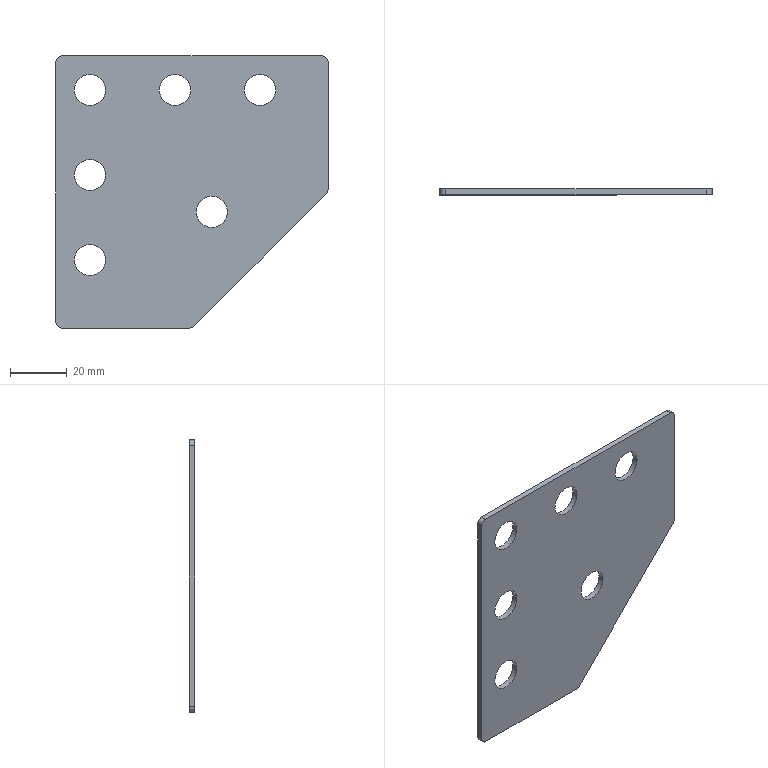Component | SolidWorks | Assembly2-1_Stiffener-2 | 1 solid | 24 faces | box 96 x 2 x 96 mm | volume 14982 mm3 | cylinder 17 | plane 7 | commonest cylinder face diameters 11 x12 4 x5
STEP:
#1=COLOUR_RGB('',0.7922,0.8196,0.9333);
#2=FILL_AREA_STYLE_COLOUR('',#1);
#3=FILL_AREA_STYLE('',(#2));
#4=SURFACE_STYLE_FILL_AREA(#3);
#5=SURFACE_SIDE_STYLE('',(#4));
#6=SURFACE_STYLE_USAGE(.BOTH.,#5);
#7=PRESENTATION_STYLE_ASSIGNMENT((#6));
#8=CARTESIAN_POINT('',(-2.167,43.439,0.3839));
#9=VERTEX_POINT('',#8);
#10=CARTESIAN_POINT('',(-1.733,43.439,0.3839));
#11=VERTEX_POINT('',#10);
#12=CARTESIAN_POINT('',(-1.95,43.439,0.3839));
#13=DIRECTION('',(-0.,1.,0.));
#14=DIRECTION('',(1.,0.,-0.));
#15=AXIS2_PLACEMENT_3D('',#12,#13,#14);
#16=CIRCLE('',#15,0.2165);
#17=EDGE_CURVE('',#9,#11,#16,.T.);
#18=ORIENTED_EDGE('',*,*,#17,.F.);
#19=CARTESIAN_POINT('',(-2.167,43.517,0.3839));
#20=VERTEX_POINT('',#19);
#21=CARTESIAN_POINT('',(-2.167,43.124,0.3839));
#22=DIRECTION('',(-0.,1.,0.));
#23=VECTOR('',#22,39.37);
#24=LINE('',#21,#23);
#25=EDGE_CURVE('',#9,#20,#24,.T.);
#26=ORIENTED_EDGE('',*,*,#25,.T.);
#27=CARTESIAN_POINT('',(-1.733,43.517,0.3839));
#28=VERTEX_POINT('',#27);
#29=CARTESIAN_POINT('',(-1.95,43.517,0.3839));
#30=DIRECTION('',(-0.,1.,0.));
#31=DIRECTION('',(1.,0.,-0.));
#32=AXIS2_PLACEMENT_3D('',#29,#30,#31);
#33=CIRCLE('',#32,0.2165);
#34=EDGE_CURVE('',#20,#28,#33,.T.);
#35=ORIENTED_EDGE('',*,*,#34,.T.);
#36=CARTESIAN_POINT('',(-1.733,43.124,0.3839));
#37=DIRECTION('',(-0.,1.,0.));
#38=VECTOR('',#37,39.37);
#39=LINE('',#36,#38);
#40=EDGE_CURVE('',#11,#28,#39,.T.);
#41=ORIENTED_EDGE('',*,*,#40,.F.);
#42=EDGE_LOOP('',(#18,#26,#35,#41));
#43=FACE_OUTER_BOUND('',#42,.T.);
#44=CARTESIAN_POINT('',(-1.95,43.124,0.3839));
#45=DIRECTION('',(-0.,1.,0.));
#46=DIRECTION('',(1.,0.,-0.));
#47=AXIS2_PLACEMENT_3D('',#44,#45,#46);
#48=CYLINDRICAL_SURFACE('',#47,0.2165);
#49=ADVANCED_FACE('',(#43),#48,.F.);
#50=CARTESIAN_POINT('',(-3.859,43.439,-0.2854));
#51=VERTEX_POINT('',#50);
#52=CARTESIAN_POINT('',(-3.426,43.439,-0.2854));
#53=VERTEX_POINT('',#52);
#54=CARTESIAN_POINT('',(-3.643,43.439,-0.2854));
#55=DIRECTION('',(-0.,1.,0.));
#56=DIRECTION('',(1.,0.,-0.));
#57=AXIS2_PLACEMENT_3D('',#54,#55,#56);
#58=CIRCLE('',#57,0.2165);
#59=EDGE_CURVE('',#51,#53,#58,.T.);
#60=ORIENTED_EDGE('',*,*,#59,.F.);
#61=CARTESIAN_POINT('',(-3.859,43.517,-0.2854));
#62=VERTEX_POINT('',#61);
#63=CARTESIAN_POINT('',(-3.859,43.124,-0.2854));
#64=DIRECTION('',(-0.,1.,0.));
#65=VECTOR('',#64,39.37);
#66=LINE('',#63,#65);
#67=EDGE_CURVE('',#51,#62,#66,.T.);
#68=ORIENTED_EDGE('',*,*,#67,.T.);
#69=CARTESIAN_POINT('',(-3.426,43.517,-0.2854));
#70=VERTEX_POINT('',#69);
#71=CARTESIAN_POINT('',(-3.643,43.517,-0.2854));
#72=DIRECTION('',(-0.,1.,0.));
#73=DIRECTION('',(1.,0.,-0.));
#74=AXIS2_PLACEMENT_3D('',#71,#72,#73);
#75=CIRCLE('',#74,0.2165);
#76=EDGE_CURVE('',#62,#70,#75,.T.);
#77=ORIENTED_EDGE('',*,*,#76,.T.);
#78=CARTESIAN_POINT('',(-3.426,43.124,-0.2854));
#79=DIRECTION('',(-0.,1.,0.));
#80=VECTOR('',#79,39.37);
#81=LINE('',#78,#80);
#82=EDGE_CURVE('',#53,#70,#81,.T.);
#83=ORIENTED_EDGE('',*,*,#82,.F.);
#84=EDGE_LOOP('',(#60,#68,#77,#83));
#85=FACE_OUTER_BOUND('',#84,.T.);
#86=CARTESIAN_POINT('',(-3.643,43.124,-0.2854));
#87=DIRECTION('',(-0.,1.,0.));
#88=DIRECTION('',(1.,0.,-0.));
#89=AXIS2_PLACEMENT_3D('',#86,#87,#88);
#90=CYLINDRICAL_SURFACE('',#89,0.2165);
#91=ADVANCED_FACE('',(#85),#90,.F.);
#92=CARTESIAN_POINT('',(-3.859,43.439,0.8957));
#93=VERTEX_POINT('',#92);
#94=CARTESIAN_POINT('',(-3.426,43.439,0.8957));
#95=VERTEX_POINT('',#94);
#96=CARTESIAN_POINT('',(-3.643,43.439,0.8957));
#97=DIRECTION('',(-0.,1.,0.));
#98=DIRECTION('',(1.,0.,-0.));
#99=AXIS2_PLACEMENT_3D('',#96,#97,#98);
#100=CIRCLE('',#99,0.2165);
#101=EDGE_CURVE('',#93,#95,#100,.T.);
#102=ORIENTED_EDGE('',*,*,#101,.F.);
#103=CARTESIAN_POINT('',(-3.859,43.517,0.8957));
#104=VERTEX_POINT('',#103);
#105=CARTESIAN_POINT('',(-3.859,43.124,0.8957));
#106=DIRECTION('',(-0.,1.,0.));
#107=VECTOR('',#106,39.37);
#108=LINE('',#105,#107);
#109=EDGE_CURVE('',#93,#104,#108,.T.);
#110=ORIENTED_EDGE('',*,*,#109,.T.);
#111=CARTESIAN_POINT('',(-3.426,43.517,0.8957));
#112=VERTEX_POINT('',#111);
#113=CARTESIAN_POINT('',(-3.643,43.517,0.8957));
#114=DIRECTION('',(-0.,1.,0.));
#115=DIRECTION('',(1.,0.,-0.));
#116=AXIS2_PLACEMENT_3D('',#113,#114,#115);
#117=CIRCLE('',#116,0.2165);
#118=EDGE_CURVE('',#104,#112,#117,.T.);
#119=ORIENTED_EDGE('',*,*,#118,.T.);
#120=CARTESIAN_POINT('',(-3.426,43.124,0.8957));
#121=DIRECTION('',(-0.,1.,0.));
#122=VECTOR('',#121,39.37);
#123=LINE('',#120,#122);
#124=EDGE_CURVE('',#95,#112,#123,.T.);
#125=ORIENTED_EDGE('',*,*,#124,.F.);
#126=EDGE_LOOP('',(#102,#110,#119,#125));
#127=FACE_OUTER_BOUND('',#126,.T.);
#128=CARTESIAN_POINT('',(-3.643,43.124,0.8957));
#129=DIRECTION('',(-0.,1.,0.));
#130=DIRECTION('',(1.,0.,-0.));
#131=AXIS2_PLACEMENT_3D('',#128,#129,#130);
#132=CYLINDRICAL_SURFACE('',#131,0.2165);
#133=ADVANCED_FACE('',(#127),#132,.F.);
#134=CARTESIAN_POINT('',(-1.497,43.439,2.077));
#135=VERTEX_POINT('',#134);
#136=CARTESIAN_POINT('',(-1.064,43.439,2.077));
#137=VERTEX_POINT('',#136);
#138=CARTESIAN_POINT('',(-1.281,43.439,2.077));
#139=DIRECTION('',(-0.,1.,0.));
#140=DIRECTION('',(1.,0.,-0.));
#141=AXIS2_PLACEMENT_3D('',#138,#139,#140);
#142=CIRCLE('',#141,0.2165);
#143=EDGE_CURVE('',#135,#137,#142,.T.);
#144=ORIENTED_EDGE('',*,*,#143,.F.);
#145=CARTESIAN_POINT('',(-1.497,43.517,2.077));
#146=VERTEX_POINT('',#145);
#147=CARTESIAN_POINT('',(-1.497,43.124,2.077));
#148=DIRECTION('',(-0.,1.,0.));
#149=VECTOR('',#148,39.37);
#150=LINE('',#147,#149);
#151=EDGE_CURVE('',#135,#146,#150,.T.);
#152=ORIENTED_EDGE('',*,*,#151,.T.);
#153=CARTESIAN_POINT('',(-1.064,43.517,2.077));
#154=VERTEX_POINT('',#153);
#155=CARTESIAN_POINT('',(-1.281,43.517,2.077));
#156=DIRECTION('',(-0.,1.,0.));
#157=DIRECTION('',(1.,0.,-0.));
#158=AXIS2_PLACEMENT_3D('',#155,#156,#157);
#159=CIRCLE('',#158,0.2165);
#160=EDGE_CURVE('',#146,#154,#159,.T.);
#161=ORIENTED_EDGE('',*,*,#160,.T.);
#162=CARTESIAN_POINT('',(-1.064,43.124,2.077));
#163=DIRECTION('',(-0.,1.,0.));
#164=VECTOR('',#163,39.37);
#165=LINE('',#162,#164);
#166=EDGE_CURVE('',#137,#154,#165,.T.);
#167=ORIENTED_EDGE('',*,*,#166,.F.);
#168=EDGE_LOOP('',(#144,#152,#161,#167));
#169=FACE_OUTER_BOUND('',#168,.T.);
#170=CARTESIAN_POINT('',(-1.281,43.124,2.077));
#171=DIRECTION('',(-0.,1.,0.));
#172=DIRECTION('',(1.,0.,-0.));
#173=AXIS2_PLACEMENT_3D('',#170,#171,#172);
#174=CYLINDRICAL_SURFACE('',#173,0.2165);
#175=ADVANCED_FACE('',(#169),#174,.F.);
#176=CARTESIAN_POINT('',(-2.678,43.439,2.077));
#177=VERTEX_POINT('',#176);
#178=CARTESIAN_POINT('',(-2.245,43.439,2.077));
#179=VERTEX_POINT('',#178);
#180=CARTESIAN_POINT('',(-2.462,43.439,2.077));
#181=DIRECTION('',(-0.,1.,0.));
#182=DIRECTION('',(1.,0.,-0.));
#183=AXIS2_PLACEMENT_3D('',#180,#181,#182);
#184=CIRCLE('',#183,0.2165);
#185=EDGE_CURVE('',#177,#179,#184,.T.);
#186=ORIENTED_EDGE('',*,*,#185,.F.);
#187=CARTESIAN_POINT('',(-2.678,43.517,2.077));
#188=VERTEX_POINT('',#187);
#189=CARTESIAN_POINT('',(-2.678,43.124,2.077));
#190=DIRECTION('',(-0.,1.,0.));
#191=VECTOR('',#190,39.37);
#192=LINE('',#189,#191);
#193=EDGE_CURVE('',#177,#188,#192,.T.);
#194=ORIENTED_EDGE('',*,*,#193,.T.);
#195=CARTESIAN_POINT('',(-2.245,43.517,2.077));
#196=VERTEX_POINT('',#195);
#197=CARTESIAN_POINT('',(-2.462,43.517,2.077));
#198=DIRECTION('',(-0.,1.,0.));
#199=DIRECTION('',(1.,0.,-0.));
#200=AXIS2_PLACEMENT_3D('',#197,#198,#199);
#201=CIRCLE('',#200,0.2165);
#202=EDGE_CURVE('',#188,#196,#201,.T.);
#203=ORIENTED_EDGE('',*,*,#202,.T.);
#204=CARTESIAN_POINT('',(-2.245,43.124,2.077));
#205=DIRECTION('',(-0.,1.,0.));
#206=VECTOR('',#205,39.37);
#207=LINE('',#204,#206);
#208=EDGE_CURVE('',#179,#196,#207,.T.);
#209=ORIENTED_EDGE('',*,*,#208,.F.);
#210=EDGE_LOOP('',(#186,#194,#203,#209));
#211=FACE_OUTER_BOUND('',#210,.T.);
#212=CARTESIAN_POINT('',(-2.462,43.124,2.077));
#213=DIRECTION('',(-0.,1.,0.));
#214=DIRECTION('',(1.,0.,-0.));
#215=AXIS2_PLACEMENT_3D('',#212,#213,#214);
#216=CYLINDRICAL_SURFACE('',#215,0.2165);
#217=ADVANCED_FACE('',(#211),#216,.F.);
#218=CARTESIAN_POINT('',(-3.859,43.439,2.077));
#219=VERTEX_POINT('',#218);
#220=CARTESIAN_POINT('',(-3.426,43.439,2.077));
#221=VERTEX_POINT('',#220);
#222=CARTESIAN_POINT('',(-3.643,43.439,2.077));
#223=DIRECTION('',(-0.,1.,0.));
#224=DIRECTION('',(1.,0.,-0.));
#225=AXIS2_PLACEMENT_3D('',#222,#223,#224);
#226=CIRCLE('',#225,0.2165);
#227=EDGE_CURVE('',#219,#221,#226,.T.);
#228=ORIENTED_EDGE('',*,*,#227,.F.);
#229=CARTESIAN_POINT('',(-3.859,43.517,2.077));
#230=VERTEX_POINT('',#229);
#231=CARTESIAN_POINT('',(-3.859,43.124,2.077));
#232=DIRECTION('',(-0.,1.,0.));
#233=VECTOR('',#232,39.37);
#234=LINE('',#231,#233);
#235=EDGE_CURVE('',#219,#230,#234,.T.);
#236=ORIENTED_EDGE('',*,*,#235,.T.);
#237=CARTESIAN_POINT('',(-3.426,43.517,2.077));
#238=VERTEX_POINT('',#237);
#239=CARTESIAN_POINT('',(-3.643,43.517,2.077));
#240=DIRECTION('',(-0.,1.,0.));
#241=DIRECTION('',(1.,0.,-0.));
#242=AXIS2_PLACEMENT_3D('',#239,#240,#241);
#243=CIRCLE('',#242,0.2165);
#244=EDGE_CURVE('',#230,#238,#243,.T.);
#245=ORIENTED_EDGE('',*,*,#244,.T.);
#246=CARTESIAN_POINT('',(-3.426,43.124,2.077));
#247=DIRECTION('',(-0.,1.,0.));
#248=VECTOR('',#247,39.37);
#249=LINE('',#246,#248);
#250=EDGE_CURVE('',#221,#238,#249,.T.);
#251=ORIENTED_EDGE('',*,*,#250,.F.);
#252=EDGE_LOOP('',(#228,#236,#245,#251));
#253=FACE_OUTER_BOUND('',#252,.T.);
#254=CARTESIAN_POINT('',(-3.643,43.124,2.077));
#255=DIRECTION('',(-0.,1.,0.));
#256=DIRECTION('',(1.,0.,-0.));
#257=AXIS2_PLACEMENT_3D('',#254,#255,#256);
#258=CYLINDRICAL_SURFACE('',#257,0.2165);
#259=ADVANCED_FACE('',(#253),#258,.F.);
#260=CARTESIAN_POINT('',(-0.3358,43.517,0.6921));
#261=VERTEX_POINT('',#260);
#262=CARTESIAN_POINT('',(-0.3589,43.517,0.6364));
#263=VERTEX_POINT('',#262);
#264=CARTESIAN_POINT('',(-0.4145,43.517,0.6921));
#265=DIRECTION('',(-0.,1.,0.));
#266=DIRECTION('',(1.,0.,-0.));
#267=AXIS2_PLACEMENT_3D('',#264,#265,#266);
#268=CIRCLE('',#267,0.07874);
#269=EDGE_CURVE('',#261,#263,#268,.T.);
#270=ORIENTED_EDGE('',*,*,#269,.F.);
#271=CARTESIAN_POINT('',(-0.3358,43.439,0.6921));
#272=VERTEX_POINT('',#271);
#273=CARTESIAN_POINT('',(-0.3358,43.439,0.6921));
#274=DIRECTION('',(-0.,1.,0.));
#275=VECTOR('',#274,39.37);
#276=LINE('',#273,#275);
#277=EDGE_CURVE('',#272,#261,#276,.T.);
#278=ORIENTED_EDGE('',*,*,#277,.F.);
#279=CARTESIAN_POINT('',(-0.3589,43.439,0.6364));
#280=VERTEX_POINT('',#279);
#281=CARTESIAN_POINT('',(-0.4145,43.439,0.6921));
#282=DIRECTION('',(-0.,1.,0.));
#283=DIRECTION('',(1.,0.,-0.));
#284=AXIS2_PLACEMENT_3D('',#281,#282,#283);
#285=CIRCLE('',#284,0.07874);
#286=EDGE_CURVE('',#272,#280,#285,.T.);
#287=ORIENTED_EDGE('',*,*,#286,.T.);
#288=CARTESIAN_POINT('',(-0.3589,43.439,0.6364));
#289=DIRECTION('',(-0.,1.,0.));
#290=VECTOR('',#289,39.37);
#291=LINE('',#288,#290);
#292=EDGE_CURVE('',#280,#263,#291,.T.);
#293=ORIENTED_EDGE('',*,*,#292,.T.);
#294=EDGE_LOOP('',(#270,#278,#287,#293));
#295=FACE_OUTER_BOUND('',#294,.T.);
#296=CARTESIAN_POINT('',(-0.4145,43.439,0.6921));
#297=DIRECTION('',(-0.,1.,0.));
#298=DIRECTION('',(1.,0.,-0.));
#299=AXIS2_PLACEMENT_3D('',#296,#297,#298);
#300=CYLINDRICAL_SURFACE('',#299,0.07874);
#301=ADVANCED_FACE('',(#295),#300,.T.);
#302=CARTESIAN_POINT('',(-0.3358,43.517,2.47));
#303=VERTEX_POINT('',#302);
#304=CARTESIAN_POINT('',(-0.3358,43.517,2.47));
#305=DIRECTION('',(-0.,0.,-1.));
#306=VECTOR('',#305,39.37);
#307=LINE('',#304,#306);
#308=EDGE_CURVE('',#303,#261,#307,.T.);
#309=ORIENTED_EDGE('',*,*,#308,.F.);
#310=CARTESIAN_POINT('',(-0.3358,43.439,2.47));
#311=VERTEX_POINT('',#310);
#312=CARTESIAN_POINT('',(-0.3358,43.439,2.47));
#313=DIRECTION('',(-0.,1.,0.));
#314=VECTOR('',#313,39.37);
#315=LINE('',#312,#314);
#316=EDGE_CURVE('',#311,#303,#315,.T.);
#317=ORIENTED_EDGE('',*,*,#316,.F.);
#318=CARTESIAN_POINT('',(-0.3358,43.439,2.47));
#319=DIRECTION('',(-0.,0.,-1.));
#320=VECTOR('',#319,39.37);
#321=LINE('',#318,#320);
#322=EDGE_CURVE('',#311,#272,#321,.T.);
#323=ORIENTED_EDGE('',*,*,#322,.T.);
#324=ORIENTED_EDGE('',*,*,#277,.T.);
#325=EDGE_LOOP('',(#309,#317,#323,#324));
#326=FACE_OUTER_BOUND('',#325,.T.);
#327=CARTESIAN_POINT('',(-0.3358,43.439,2.47));
#328=DIRECTION('',(1.,0.,-0.));
#329=DIRECTION('',(0.,-1.,-0.));
#330=AXIS2_PLACEMENT_3D('',#327,#328,#329);
#331=PLANE('',#330);
#332=ADVANCED_FACE('',(#326),#331,.T.);
#333=CARTESIAN_POINT('',(-0.4145,43.517,2.549));
#334=VERTEX_POINT('',#333);
#335=CARTESIAN_POINT('',(-0.4145,43.517,2.47));
#336=DIRECTION('',(-0.,1.,0.));
#337=DIRECTION('',(1.,0.,0.));
#338=AXIS2_PLACEMENT_3D('',#335,#336,#337);
#339=CIRCLE('',#338,0.07874);
#340=EDGE_CURVE('',#334,#303,#339,.T.);
#341=ORIENTED_EDGE('',*,*,#340,.F.);
#342=CARTESIAN_POINT('',(-0.4145,43.439,2.549));
#343=VERTEX_POINT('',#342);
#344=CARTESIAN_POINT('',(-0.4145,43.439,2.549));
#345=DIRECTION('',(-0.,1.,0.));
#346=VECTOR('',#345,39.37);
#347=LINE('',#344,#346);
#348=EDGE_CURVE('',#343,#334,#347,.T.);
#349=ORIENTED_EDGE('',*,*,#348,.F.);
#350=CARTESIAN_POINT('',(-0.4145,43.439,2.47));
#351=DIRECTION('',(-0.,1.,0.));
#352=DIRECTION('',(1.,0.,0.));
#353=AXIS2_PLACEMENT_3D('',#350,#351,#352);
#354=CIRCLE('',#353,0.07874);
#355=EDGE_CURVE('',#343,#311,#354,.T.);
#356=ORIENTED_EDGE('',*,*,#355,.T.);
#357=ORIENTED_EDGE('',*,*,#316,.T.);
#358=EDGE_LOOP('',(#341,#349,#356,#357));
#359=FACE_OUTER_BOUND('',#358,.T.);
#360=CARTESIAN_POINT('',(-0.4145,43.439,2.47));
#361=DIRECTION('',(-0.,1.,0.));
#362=DIRECTION('',(1.,0.,0.));
#363=AXIS2_PLACEMENT_3D('',#360,#361,#362);
#364=CYLINDRICAL_SURFACE('',#363,0.07874);
#365=ADVANCED_FACE('',(#359),#364,.T.);
#366=CARTESIAN_POINT('',(-4.037,43.517,2.549));
#367=VERTEX_POINT('',#366);
#368=CARTESIAN_POINT('',(-4.037,43.517,2.549));
#369=DIRECTION('',(1.,0.,-0.));
#370=VECTOR('',#369,39.37);
#371=LINE('',#368,#370);
#372=EDGE_CURVE('',#367,#334,#371,.T.);
#373=ORIENTED_EDGE('',*,*,#372,.F.);
#374=CARTESIAN_POINT('',(-4.037,43.439,2.549));
#375=VERTEX_POINT('',#374);
#376=CARTESIAN_POINT('',(-4.037,43.439,2.549));
#377=DIRECTION('',(-0.,1.,0.));
#378=VECTOR('',#377,39.37);
#379=LINE('',#376,#378);
#380=EDGE_CURVE('',#375,#367,#379,.T.);
#381=ORIENTED_EDGE('',*,*,#380,.F.);
#382=CARTESIAN_POINT('',(-4.037,43.439,2.549));
#383=DIRECTION('',(1.,0.,-0.));
#384=VECTOR('',#383,39.37);
#385=LINE('',#382,#384);
#386=EDGE_CURVE('',#375,#343,#385,.T.);
#387=ORIENTED_EDGE('',*,*,#386,.T.);
#388=ORIENTED_EDGE('',*,*,#348,.T.);
#389=EDGE_LOOP('',(#373,#381,#387,#388));
#390=FACE_OUTER_BOUND('',#389,.T.);
#391=CARTESIAN_POINT('',(-4.037,43.439,2.549));
#392=DIRECTION('',(0.,-0.,1.));
#393=DIRECTION('',(0.,-1.,-0.));
#394=AXIS2_PLACEMENT_3D('',#391,#392,#393);
#395=PLANE('',#394);
#396=ADVANCED_FACE('',(#390),#395,.T.);
#397=CARTESIAN_POINT('',(-4.115,43.517,2.47));
#398=VERTEX_POINT('',#397);
#399=CARTESIAN_POINT('',(-4.037,43.517,2.47));
#400=DIRECTION('',(-0.,1.,0.));
#401=DIRECTION('',(-1.,0.,0.));
#402=AXIS2_PLACEMENT_3D('',#399,#400,#401);
#403=CIRCLE('',#402,0.07874);
#404=EDGE_CURVE('',#398,#367,#403,.T.);
#405=ORIENTED_EDGE('',*,*,#404,.F.);
#406=CARTESIAN_POINT('',(-4.115,43.439,2.47));
#407=VERTEX_POINT('',#406);
#408=CARTESIAN_POINT('',(-4.115,43.439,2.47));
#409=DIRECTION('',(-0.,1.,0.));
#410=VECTOR('',#409,39.37);
#411=LINE('',#408,#410);
#412=EDGE_CURVE('',#407,#398,#411,.T.);
#413=ORIENTED_EDGE('',*,*,#412,.F.);
#414=CARTESIAN_POINT('',(-4.037,43.439,2.47));
#415=DIRECTION('',(-0.,1.,0.));
#416=DIRECTION('',(-1.,0.,0.));
#417=AXIS2_PLACEMENT_3D('',#414,#415,#416);
#418=CIRCLE('',#417,0.07874);
#419=EDGE_CURVE('',#407,#375,#418,.T.);
#420=ORIENTED_EDGE('',*,*,#419,.T.);
#421=ORIENTED_EDGE('',*,*,#380,.T.);
#422=EDGE_LOOP('',(#405,#413,#420,#421));
#423=FACE_OUTER_BOUND('',#422,.T.);
#424=CARTESIAN_POINT('',(-4.037,43.439,2.47));
#425=DIRECTION('',(-0.,1.,0.));
#426=DIRECTION('',(1.,0.,0.));
#427=AXIS2_PLACEMENT_3D('',#424,#425,#426);
#428=CYLINDRICAL_SURFACE('',#427,0.07874);
#429=ADVANCED_FACE('',(#423),#428,.T.);
#430=CARTESIAN_POINT('',(-4.115,43.517,-1.152));
#431=VERTEX_POINT('',#430);
#432=CARTESIAN_POINT('',(-4.115,43.517,2.47));
#433=DIRECTION('',(0.,-0.,1.));
#434=VECTOR('',#433,39.37);
#435=LINE('',#432,#434);
#436=EDGE_CURVE('',#431,#398,#435,.T.);
#437=ORIENTED_EDGE('',*,*,#436,.F.);
#438=CARTESIAN_POINT('',(-4.115,43.439,-1.152));
#439=VERTEX_POINT('',#438);
#440=CARTESIAN_POINT('',(-4.115,43.439,-1.152));
#441=DIRECTION('',(-0.,1.,0.));
#442=VECTOR('',#441,39.37);
#443=LINE('',#440,#442);
#444=EDGE_CURVE('',#439,#431,#443,.T.);
#445=ORIENTED_EDGE('',*,*,#444,.F.);
#446=CARTESIAN_POINT('',(-4.115,43.439,2.47));
#447=DIRECTION('',(0.,-0.,1.));
#448=VECTOR('',#447,39.37);
#449=LINE('',#446,#448);
#450=EDGE_CURVE('',#439,#407,#449,.T.);
#451=ORIENTED_EDGE('',*,*,#450,.T.);
#452=ORIENTED_EDGE('',*,*,#412,.T.);
#453=EDGE_LOOP('',(#437,#445,#451,#452));
#454=FACE_OUTER_BOUND('',#453,.T.);
#455=CARTESIAN_POINT('',(-4.115,43.439,2.47));
#456=DIRECTION('',(-1.,-0.,0.));
#457=DIRECTION('',(-0.,1.,0.));
#458=AXIS2_PLACEMENT_3D('',#455,#456,#457);
#459=PLANE('',#458);
#460=ADVANCED_FACE('',(#454),#459,.T.);
#461=CARTESIAN_POINT('',(-4.037,43.517,-1.23));
#462=VERTEX_POINT('',#461);
#463=CARTESIAN_POINT('',(-4.037,43.517,-1.152));
#464=DIRECTION('',(-0.,1.,0.));
#465=DIRECTION('',(-1.,0.,0.));
#466=AXIS2_PLACEMENT_3D('',#463,#464,#465);
#467=CIRCLE('',#466,0.07874);
#468=EDGE_CURVE('',#462,#431,#467,.T.);
#469=ORIENTED_EDGE('',*,*,#468,.F.);
#470=CARTESIAN_POINT('',(-4.037,43.439,-1.23));
#471=VERTEX_POINT('',#470);
#472=CARTESIAN_POINT('',(-4.037,43.439,-1.23));
#473=DIRECTION('',(-0.,1.,0.));
#474=VECTOR('',#473,39.37);
#475=LINE('',#472,#474);
#476=EDGE_CURVE('',#471,#462,#475,.T.);
#477=ORIENTED_EDGE('',*,*,#476,.F.);
#478=CARTESIAN_POINT('',(-4.037,43.439,-1.152));
#479=DIRECTION('',(-0.,1.,0.));
#480=DIRECTION('',(-1.,0.,0.));
#481=AXIS2_PLACEMENT_3D('',#478,#479,#480);
#482=CIRCLE('',#481,0.07874);
#483=EDGE_CURVE('',#471,#439,#482,.T.);
#484=ORIENTED_EDGE('',*,*,#483,.T.);
#485=ORIENTED_EDGE('',*,*,#444,.T.);
#486=EDGE_LOOP('',(#469,#477,#484,#485));
#487=FACE_OUTER_BOUND('',#486,.T.);
#488=CARTESIAN_POINT('',(-4.037,43.439,-1.152));
#489=DIRECTION('',(-0.,1.,0.));
#490=DIRECTION('',(1.,0.,-0.));
#491=AXIS2_PLACEMENT_3D('',#488,#489,#490);
#492=CYLINDRICAL_SURFACE('',#491,0.07874);
#493=ADVANCED_FACE('',(#487),#492,.T.);
#494=CARTESIAN_POINT('',(-2.258,43.517,-1.23));
#495=VERTEX_POINT('',#494);
#496=CARTESIAN_POINT('',(-4.037,43.517,-1.23));
#497=DIRECTION('',(-1.,-0.,0.));
#498=VECTOR('',#497,39.37);
#499=LINE('',#496,#498);
#500=EDGE_CURVE('',#495,#462,#499,.T.);
#501=ORIENTED_EDGE('',*,*,#500,.F.);
#502=CARTESIAN_POINT('',(-2.258,43.439,-1.23));
#503=VERTEX_POINT('',#502);
#504=CARTESIAN_POINT('',(-2.258,43.439,-1.23));
#505=DIRECTION('',(-0.,1.,0.));
#506=VECTOR('',#505,39.37);
#507=LINE('',#504,#506);
#508=EDGE_CURVE('',#503,#495,#507,.T.);
#509=ORIENTED_EDGE('',*,*,#508,.F.);
#510=CARTESIAN_POINT('',(-4.037,43.439,-1.23));
#511=DIRECTION('',(-1.,-0.,0.));
#512=VECTOR('',#511,39.37);
#513=LINE('',#510,#512);
#514=EDGE_CURVE('',#503,#471,#513,.T.);
#515=ORIENTED_EDGE('',*,*,#514,.T.);
#516=ORIENTED_EDGE('',*,*,#476,.T.);
#517=EDGE_LOOP('',(#501,#509,#515,#516));
#518=FACE_OUTER_BOUND('',#517,.T.);
#519=CARTESIAN_POINT('',(-4.037,43.439,-1.23));
#520=DIRECTION('',(-0.,0.,-1.));
#521=DIRECTION('',(-0.,1.,0.));
#522=AXIS2_PLACEMENT_3D('',#519,#520,#521);
#523=PLANE('',#522);
#524=ADVANCED_FACE('',(#518),#523,.T.);
#525=CARTESIAN_POINT('',(-2.202,43.517,-1.207));
#526=VERTEX_POINT('',#525);
#527=CARTESIAN_POINT('',(-2.258,43.517,-1.152));
#528=DIRECTION('',(-0.,1.,0.));
#529=DIRECTION('',(1.,0.,-0.));
#530=AXIS2_PLACEMENT_3D('',#527,#528,#529);
#531=CIRCLE('',#530,0.07874);
#532=EDGE_CURVE('',#526,#495,#531,.T.);
#533=ORIENTED_EDGE('',*,*,#532,.F.);
#534=CARTESIAN_POINT('',(-2.202,43.439,-1.207));
#535=VERTEX_POINT('',#534);
#536=CARTESIAN_POINT('',(-2.202,43.439,-1.207));
#537=DIRECTION('',(-0.,1.,0.));
#538=VECTOR('',#537,39.37);
#539=LINE('',#536,#538);
#540=EDGE_CURVE('',#535,#526,#539,.T.);
#541=ORIENTED_EDGE('',*,*,#540,.F.);
#542=CARTESIAN_POINT('',(-2.258,43.439,-1.152));
#543=DIRECTION('',(-0.,1.,0.));
#544=DIRECTION('',(1.,0.,-0.));
#545=AXIS2_PLACEMENT_3D('',#542,#543,#544);
#546=CIRCLE('',#545,0.07874);
#547=EDGE_CURVE('',#535,#503,#546,.T.);
#548=ORIENTED_EDGE('',*,*,#547,.T.);
#549=ORIENTED_EDGE('',*,*,#508,.T.);
#550=EDGE_LOOP('',(#533,#541,#548,#549));
#551=FACE_OUTER_BOUND('',#550,.T.);
#552=CARTESIAN_POINT('',(-2.258,43.439,-1.152));
#553=DIRECTION('',(-0.,1.,0.));
#554=DIRECTION('',(1.,0.,-0.));
#555=AXIS2_PLACEMENT_3D('',#552,#553,#554);
#556=CYLINDRICAL_SURFACE('',#555,0.07874);
#557=ADVANCED_FACE('',(#551),#556,.T.);
#558=CARTESIAN_POINT('',(-2.202,43.517,-1.207));
#559=DIRECTION('',(-0.7071,-0.,-0.7071));
#560=VECTOR('',#559,39.37);
#561=LINE('',#558,#560);
#562=EDGE_CURVE('',#263,#526,#561,.T.);
#563=ORIENTED_EDGE('',*,*,#562,.F.);
#564=ORIENTED_EDGE('',*,*,#292,.F.);
#565=CARTESIAN_POINT('',(-2.202,43.439,-1.207));
#566=DIRECTION('',(-0.7071,-0.,-0.7071));
#567=VECTOR('',#566,39.37);
#568=LINE('',#565,#567);
#569=EDGE_CURVE('',#280,#535,#568,.T.);
#570=ORIENTED_EDGE('',*,*,#569,.T.);
#571=ORIENTED_EDGE('',*,*,#540,.T.);
#572=EDGE_LOOP('',(#563,#564,#570,#571));
#573=FACE_OUTER_BOUND('',#572,.T.);
#574=CARTESIAN_POINT('',(-2.202,43.439,-1.207));
#575=DIRECTION('',(0.7071,0.,-0.7071));
#576=DIRECTION('',(-0.7071,-0.,-0.7071));
#577=AXIS2_PLACEMENT_3D('',#574,#575,#576);
#578=PLANE('',#577);
#579=ADVANCED_FACE('',(#573),#578,.T.);
#580=CARTESIAN_POINT('',(-1.95,43.439,0.3839));
#581=DIRECTION('',(-0.,1.,0.));
#582=DIRECTION('',(1.,0.,-0.));
#583=AXIS2_PLACEMENT_3D('',#580,#581,#582);
#584=CIRCLE('',#583,0.2165);
#585=EDGE_CURVE('',#11,#9,#584,.T.);
#586=ORIENTED_EDGE('',*,*,#585,.T.);
#587=ORIENTED_EDGE('',*,*,#17,.T.);
#588=EDGE_LOOP('',(#586,#587));
#589=FACE_BOUND('',#588,.T.);
#590=CARTESIAN_POINT('',(-3.643,43.439,-0.2854));
#591=DIRECTION('',(-0.,1.,0.));
#592=DIRECTION('',(1.,0.,-0.));
#593=AXIS2_PLACEMENT_3D('',#590,#591,#592);
#594=CIRCLE('',#593,0.2165);
#595=EDGE_CURVE('',#53,#51,#594,.T.);
#596=ORIENTED_EDGE('',*,*,#595,.T.);
#597=ORIENTED_EDGE('',*,*,#59,.T.);
#598=EDGE_LOOP('',(#596,#597));
#599=FACE_BOUND('',#598,.T.);
#600=CARTESIAN_POINT('',(-3.643,43.439,0.8957));
#601=DIRECTION('',(-0.,1.,0.));
#602=DIRECTION('',(1.,0.,-0.));
#603=AXIS2_PLACEMENT_3D('',#600,#601,#602);
#604=CIRCLE('',#603,0.2165);
#605=EDGE_CURVE('',#95,#93,#604,.T.);
#606=ORIENTED_EDGE('',*,*,#605,.T.);
#607=ORIENTED_EDGE('',*,*,#101,.T.);
#608=EDGE_LOOP('',(#606,#607));
#609=FACE_BOUND('',#608,.T.);
#610=CARTESIAN_POINT('',(-1.281,43.439,2.077));
#611=DIRECTION('',(-0.,1.,0.));
#612=DIRECTION('',(1.,0.,-0.));
#613=AXIS2_PLACEMENT_3D('',#610,#611,#612);
#614=CIRCLE('',#613,0.2165);
#615=EDGE_CURVE('',#137,#135,#614,.T.);
#616=ORIENTED_EDGE('',*,*,#615,.T.);
#617=ORIENTED_EDGE('',*,*,#143,.T.);
#618=EDGE_LOOP('',(#616,#617));
#619=FACE_BOUND('',#618,.T.);
#620=CARTESIAN_POINT('',(-2.462,43.439,2.077));
#621=DIRECTION('',(-0.,1.,0.));
#622=DIRECTION('',(1.,0.,-0.));
#623=AXIS2_PLACEMENT_3D('',#620,#621,#622);
#624=CIRCLE('',#623,0.2165);
#625=EDGE_CURVE('',#179,#177,#624,.T.);
#626=ORIENTED_EDGE('',*,*,#625,.T.);
#627=ORIENTED_EDGE('',*,*,#185,.T.);
#628=EDGE_LOOP('',(#626,#627));
#629=FACE_BOUND('',#628,.T.);
#630=CARTESIAN_POINT('',(-3.643,43.439,2.077));
#631=DIRECTION('',(-0.,1.,0.));
#632=DIRECTION('',(1.,0.,-0.));
#633=AXIS2_PLACEMENT_3D('',#630,#631,#632);
#634=CIRCLE('',#633,0.2165);
#635=EDGE_CURVE('',#221,#219,#634,.T.);
#636=ORIENTED_EDGE('',*,*,#635,.T.);
#637=ORIENTED_EDGE('',*,*,#227,.T.);
#638=EDGE_LOOP('',(#636,#637));
#639=FACE_BOUND('',#638,.T.);
#640=ORIENTED_EDGE('',*,*,#286,.F.);
#641=ORIENTED_EDGE('',*,*,#322,.F.);
#642=ORIENTED_EDGE('',*,*,#355,.F.);
#643=ORIENTED_EDGE('',*,*,#386,.F.);
#644=ORIENTED_EDGE('',*,*,#419,.F.);
#645=ORIENTED_EDGE('',*,*,#450,.F.);
#646=ORIENTED_EDGE('',*,*,#483,.F.);
#647=ORIENTED_EDGE('',*,*,#514,.F.);
#648=ORIENTED_EDGE('',*,*,#547,.F.);
#649=ORIENTED_EDGE('',*,*,#569,.F.);
#650=EDGE_LOOP('',(#640,#641,#642,#643,#644,#645,#646,#647,#648,#649));
#651=FACE_OUTER_BOUND('',#650,.T.);
#652=CARTESIAN_POINT('',(-0.4145,43.439,0.6921));
#653=DIRECTION('',(-0.,1.,0.));
#654=DIRECTION('',(1.,0.,-0.));
#655=AXIS2_PLACEMENT_3D('',#652,#653,#654);
#656=PLANE('',#655);
#657=ADVANCED_FACE('',(#589,#599,#609,#619,#629,#639,#651),#656,.F.);
#658=CARTESIAN_POINT('',(-1.95,43.517,0.3839));
#659=DIRECTION('',(-0.,1.,0.));
#660=DIRECTION('',(1.,0.,-0.));
#661=AXIS2_PLACEMENT_3D('',#658,#659,#660);
#662=CIRCLE('',#661,0.2165);
#663=EDGE_CURVE('',#28,#20,#662,.T.);
#664=ORIENTED_EDGE('',*,*,#663,.F.);
#665=ORIENTED_EDGE('',*,*,#34,.F.);
#666=EDGE_LOOP('',(#664,#665));
#667=FACE_BOUND('',#666,.T.);
#668=CARTESIAN_POINT('',(-3.643,43.517,-0.2854));
#669=DIRECTION('',(-0.,1.,0.));
#670=DIRECTION('',(1.,0.,-0.));
#671=AXIS2_PLACEMENT_3D('',#668,#669,#670);
#672=CIRCLE('',#671,0.2165);
#673=EDGE_CURVE('',#70,#62,#672,.T.);
#674=ORIENTED_EDGE('',*,*,#673,.F.);
#675=ORIENTED_EDGE('',*,*,#76,.F.);
#676=EDGE_LOOP('',(#674,#675));
#677=FACE_BOUND('',#676,.T.);
#678=CARTESIAN_POINT('',(-3.643,43.517,0.8957));
#679=DIRECTION('',(-0.,1.,0.));
#680=DIRECTION('',(1.,0.,-0.));
#681=AXIS2_PLACEMENT_3D('',#678,#679,#680);
#682=CIRCLE('',#681,0.2165);
#683=EDGE_CURVE('',#112,#104,#682,.T.);
#684=ORIENTED_EDGE('',*,*,#683,.F.);
#685=ORIENTED_EDGE('',*,*,#118,.F.);
#686=EDGE_LOOP('',(#684,#685));
#687=FACE_BOUND('',#686,.T.);
#688=CARTESIAN_POINT('',(-1.281,43.517,2.077));
#689=DIRECTION('',(-0.,1.,0.));
#690=DIRECTION('',(1.,0.,-0.));
#691=AXIS2_PLACEMENT_3D('',#688,#689,#690);
#692=CIRCLE('',#691,0.2165);
#693=EDGE_CURVE('',#154,#146,#692,.T.);
#694=ORIENTED_EDGE('',*,*,#693,.F.);
#695=ORIENTED_EDGE('',*,*,#160,.F.);
#696=EDGE_LOOP('',(#694,#695));
#697=FACE_BOUND('',#696,.T.);
#698=CARTESIAN_POINT('',(-2.462,43.517,2.077));
#699=DIRECTION('',(-0.,1.,0.));
#700=DIRECTION('',(1.,0.,-0.));
#701=AXIS2_PLACEMENT_3D('',#698,#699,#700);
#702=CIRCLE('',#701,0.2165);
#703=EDGE_CURVE('',#196,#188,#702,.T.);
#704=ORIENTED_EDGE('',*,*,#703,.F.);
#705=ORIENTED_EDGE('',*,*,#202,.F.);
#706=EDGE_LOOP('',(#704,#705));
#707=FACE_BOUND('',#706,.T.);
#708=CARTESIAN_POINT('',(-3.643,43.517,2.077));
#709=DIRECTION('',(-0.,1.,0.));
#710=DIRECTION('',(1.,0.,-0.));
#711=AXIS2_PLACEMENT_3D('',#708,#709,#710);
#712=CIRCLE('',#711,0.2165);
#713=EDGE_CURVE('',#238,#230,#712,.T.);
#714=ORIENTED_EDGE('',*,*,#713,.F.);
#715=ORIENTED_EDGE('',*,*,#244,.F.);
#716=EDGE_LOOP('',(#714,#715));
#717=FACE_BOUND('',#716,.T.);
#718=ORIENTED_EDGE('',*,*,#269,.T.);
#719=ORIENTED_EDGE('',*,*,#562,.T.);
#720=ORIENTED_EDGE('',*,*,#532,.T.);
#721=ORIENTED_EDGE('',*,*,#500,.T.);
#722=ORIENTED_EDGE('',*,*,#468,.T.);
#723=ORIENTED_EDGE('',*,*,#436,.T.);
#724=ORIENTED_EDGE('',*,*,#404,.T.);
#725=ORIENTED_EDGE('',*,*,#372,.T.);
#726=ORIENTED_EDGE('',*,*,#340,.T.);
#727=ORIENTED_EDGE('',*,*,#308,.T.);
#728=EDGE_LOOP('',(#718,#719,#720,#721,#722,#723,#724,#725,#726,#727));
#729=FACE_OUTER_BOUND('',#728,.T.);
#730=CARTESIAN_POINT('',(-0.4145,43.517,0.6921));
#731=DIRECTION('',(-0.,1.,0.));
#732=DIRECTION('',(1.,0.,-0.));
#733=AXIS2_PLACEMENT_3D('',#730,#731,#732);
#734=PLANE('',#733);
#735=ADVANCED_FACE('',(#667,#677,#687,#697,#707,#717,#729),#734,.T.);
#736=ORIENTED_EDGE('',*,*,#235,.F.);
#737=ORIENTED_EDGE('',*,*,#635,.F.);
#738=ORIENTED_EDGE('',*,*,#250,.T.);
#739=ORIENTED_EDGE('',*,*,#713,.T.);
#740=EDGE_LOOP('',(#736,#737,#738,#739));
#741=FACE_OUTER_BOUND('',#740,.T.);
#742=CARTESIAN_POINT('',(-3.643,43.124,2.077));
#743=DIRECTION('',(-0.,1.,0.));
#744=DIRECTION('',(1.,0.,-0.));
#745=AXIS2_PLACEMENT_3D('',#742,#743,#744);
#746=CYLINDRICAL_SURFACE('',#745,0.2165);
#747=ADVANCED_FACE('',(#741),#746,.F.);
#748=ORIENTED_EDGE('',*,*,#193,.F.);
#749=ORIENTED_EDGE('',*,*,#625,.F.);
#750=ORIENTED_EDGE('',*,*,#208,.T.);
#751=ORIENTED_EDGE('',*,*,#703,.T.);
#752=EDGE_LOOP('',(#748,#749,#750,#751));
#753=FACE_OUTER_BOUND('',#752,.T.);
#754=CARTESIAN_POINT('',(-2.462,43.124,2.077));
#755=DIRECTION('',(-0.,1.,0.));
#756=DIRECTION('',(1.,0.,-0.));
#757=AXIS2_PLACEMENT_3D('',#754,#755,#756);
#758=CYLINDRICAL_SURFACE('',#757,0.2165);
#759=ADVANCED_FACE('',(#753),#758,.F.);
#760=ORIENTED_EDGE('',*,*,#151,.F.);
#761=ORIENTED_EDGE('',*,*,#615,.F.);
#762=ORIENTED_EDGE('',*,*,#166,.T.);
#763=ORIENTED_EDGE('',*,*,#693,.T.);
#764=EDGE_LOOP('',(#760,#761,#762,#763));
#765=FACE_OUTER_BOUND('',#764,.T.);
#766=CARTESIAN_POINT('',(-1.281,43.124,2.077));
#767=DIRECTION('',(-0.,1.,0.));
#768=DIRECTION('',(1.,0.,-0.));
#769=AXIS2_PLACEMENT_3D('',#766,#767,#768);
#770=CYLINDRICAL_SURFACE('',#769,0.2165);
#771=ADVANCED_FACE('',(#765),#770,.F.);
#772=ORIENTED_EDGE('',*,*,#109,.F.);
#773=ORIENTED_EDGE('',*,*,#605,.F.);
#774=ORIENTED_EDGE('',*,*,#124,.T.);
#775=ORIENTED_EDGE('',*,*,#683,.T.);
#776=EDGE_LOOP('',(#772,#773,#774,#775));
#777=FACE_OUTER_BOUND('',#776,.T.);
#778=CARTESIAN_POINT('',(-3.643,43.124,0.8957));
#779=DIRECTION('',(-0.,1.,0.));
#780=DIRECTION('',(1.,0.,-0.));
#781=AXIS2_PLACEMENT_3D('',#778,#779,#780);
#782=CYLINDRICAL_SURFACE('',#781,0.2165);
#783=ADVANCED_FACE('',(#777),#782,.F.);
#784=ORIENTED_EDGE('',*,*,#67,.F.);
#785=ORIENTED_EDGE('',*,*,#595,.F.);
#786=ORIENTED_EDGE('',*,*,#82,.T.);
#787=ORIENTED_EDGE('',*,*,#673,.T.);
#788=EDGE_LOOP('',(#784,#785,#786,#787));
#789=FACE_OUTER_BOUND('',#788,.T.);
#790=CARTESIAN_POINT('',(-3.643,43.124,-0.2854));
#791=DIRECTION('',(-0.,1.,0.));
#792=DIRECTION('',(1.,0.,-0.));
#793=AXIS2_PLACEMENT_3D('',#790,#791,#792);
#794=CYLINDRICAL_SURFACE('',#793,0.2165);
#795=ADVANCED_FACE('',(#789),#794,.F.);
#796=ORIENTED_EDGE('',*,*,#25,.F.);
#797=ORIENTED_EDGE('',*,*,#585,.F.);
#798=ORIENTED_EDGE('',*,*,#40,.T.);
#799=ORIENTED_EDGE('',*,*,#663,.T.);
#800=EDGE_LOOP('',(#796,#797,#798,#799));
#801=FACE_OUTER_BOUND('',#800,.T.);
#802=CARTESIAN_POINT('',(-1.95,43.124,0.3839));
#803=DIRECTION('',(-0.,1.,0.));
#804=DIRECTION('',(1.,0.,-0.));
#805=AXIS2_PLACEMENT_3D('',#802,#803,#804);
#806=CYLINDRICAL_SURFACE('',#805,0.2165);
#807=ADVANCED_FACE('',(#801),#806,.F.);
#808=CLOSED_SHELL('',(#49,#91,#133,#175,#217,#259,#301,#332,#365,#396,#429,#460,#493,#524,#557,#579,#657,#735,#747,#759,#771,#783,#795,#807));
#809=MANIFOLD_SOLID_BREP('',#808);
#810=STYLED_ITEM('',(#7),#809);
#811=PRESENTATION_LAYER_ASSIGNMENT('','',(#810));
#812=(LENGTH_UNIT()NAMED_UNIT(*)SI_UNIT($,.METRE.));
#813=LENGTH_MEASURE_WITH_UNIT(LENGTH_MEASURE(0.0254),#812);
#814=DIMENSIONAL_EXPONENTS(1.,0.,0.,0.,0.,0.,0.);
#815=(CONVERSION_BASED_UNIT('',#813)LENGTH_UNIT()NAMED_UNIT(#814));
#816=UNCERTAINTY_MEASURE_WITH_UNIT(LENGTH_MEASURE(0.00001),#815,'','');
#817=(NAMED_UNIT(*)PLANE_ANGLE_UNIT()SI_UNIT($,.RADIAN.));
#818=(NAMED_UNIT(*)SI_UNIT($,.STERADIAN.)SOLID_ANGLE_UNIT());
#819=(GEOMETRIC_REPRESENTATION_CONTEXT(3)GLOBAL_UNCERTAINTY_ASSIGNED_CONTEXT((#816))GLOBAL_UNIT_ASSIGNED_CONTEXT((#815,#817,#818))REPRESENTATION_CONTEXT('',''));
#820=MECHANICAL_DESIGN_GEOMETRIC_PRESENTATION_REPRESENTATION('',(#810),#819);
#821=CARTESIAN_POINT('',(0.,0.,0.));
#822=DIRECTION('',(0.,0.,1.));
#823=DIRECTION('',(1.,0.,0.));
#824=AXIS2_PLACEMENT_3D('',#821,#822,#823);
#825=(LENGTH_UNIT()NAMED_UNIT(*)SI_UNIT($,.METRE.));
#826=LENGTH_MEASURE_WITH_UNIT(LENGTH_MEASURE(0.0254),#825);
#827=DIMENSIONAL_EXPONENTS(1.,0.,0.,0.,0.,0.,0.);
#828=(CONVERSION_BASED_UNIT('',#826)LENGTH_UNIT()NAMED_UNIT(#827));
#829=UNCERTAINTY_MEASURE_WITH_UNIT(LENGTH_MEASURE(0.00001),#828,'','');
#830=(NAMED_UNIT(*)PLANE_ANGLE_UNIT()SI_UNIT($,.RADIAN.));
#831=(NAMED_UNIT(*)SI_UNIT($,.STERADIAN.)SOLID_ANGLE_UNIT());
#832=(GEOMETRIC_REPRESENTATION_CONTEXT(3)GLOBAL_UNCERTAINTY_ASSIGNED_CONTEXT((#829))GLOBAL_UNIT_ASSIGNED_CONTEXT((#828,#830,#831))REPRESENTATION_CONTEXT('',''));
#833=ADVANCED_BREP_SHAPE_REPRESENTATION('',(#809,#824),#832);